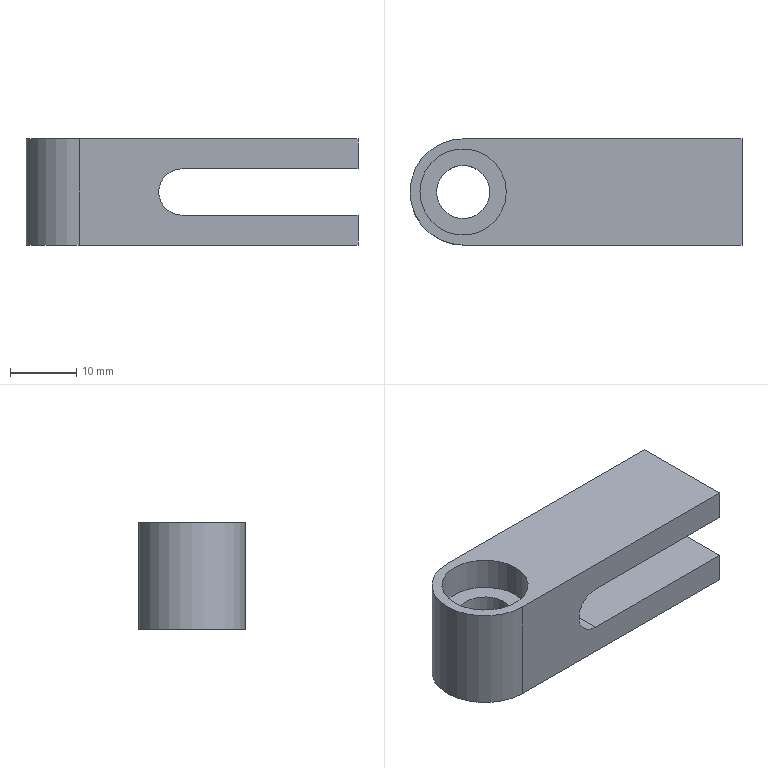CAM job | Mastercam | mm | 13 operations | part box 50 x 16 x 16
1. Facing | 24 - 100 平铣刀
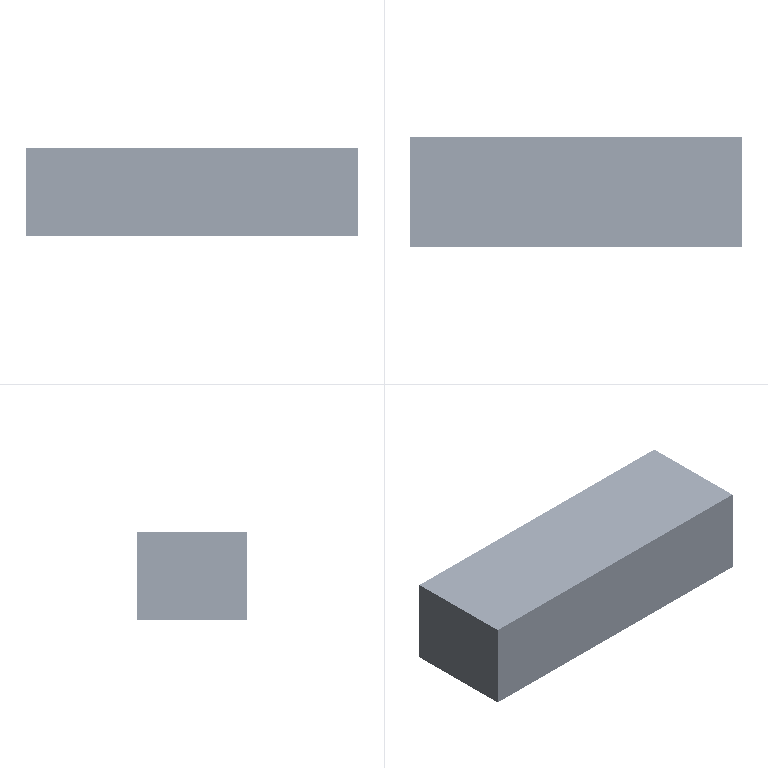2. Contour (Ramp) | 9 - 10 平铣刀
3. Contour (2D) | 10 - 10 平铣刀
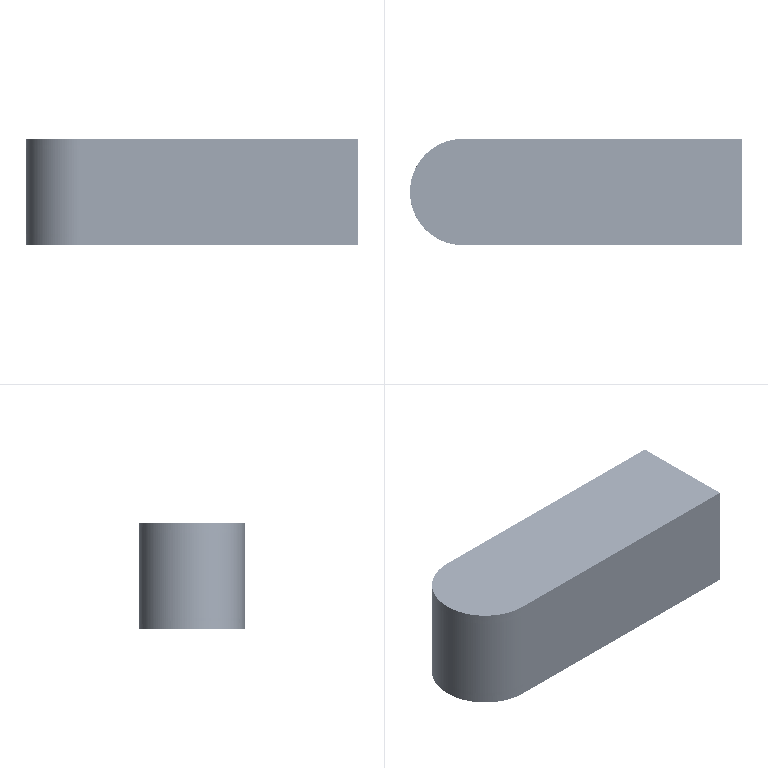4. Drill/Counterbore | 5 - 4 倒角刀
5. Peck Drill | 1 - 8 钻头
6. Contour (Ramp) | 6 - 6 平铣刀
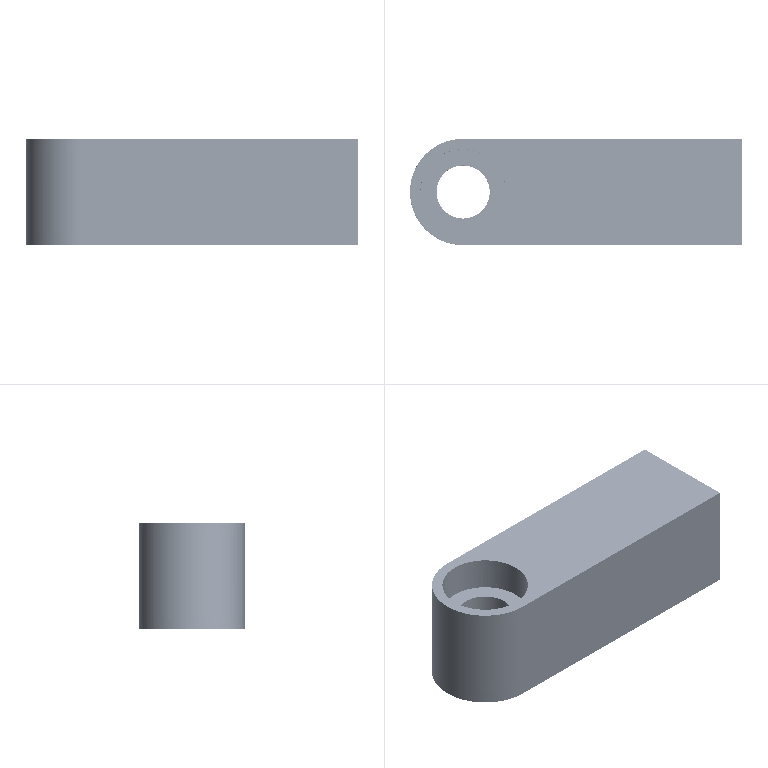7. Contour (2D) | 6 - 6 平铣刀
8. Contour (2D chamfer) | 5 - 4 倒角刀
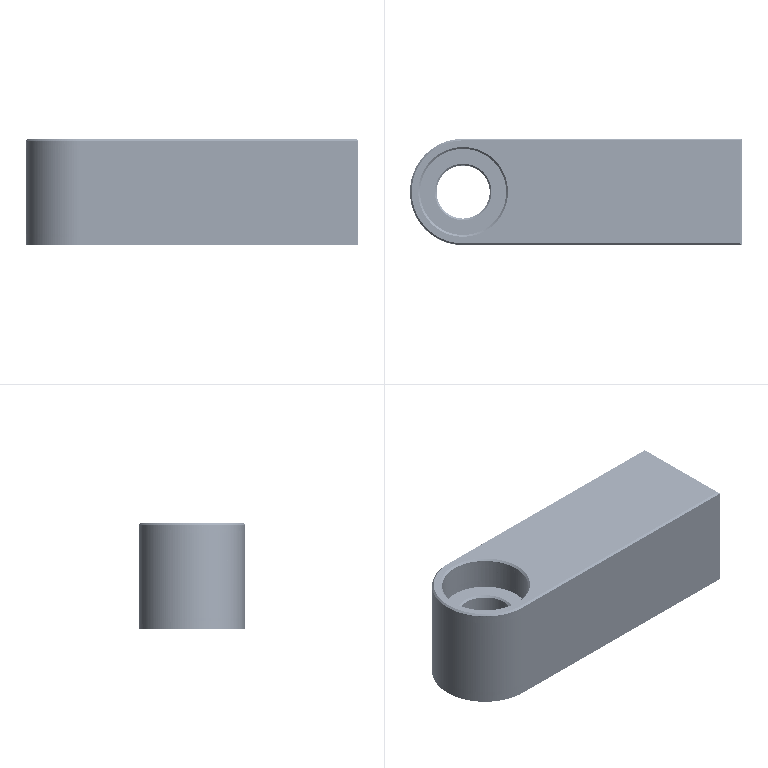9. Facing | 24 - 100 平铣刀
10. Contour (2D chamfer) | 5 - 4 倒角刀
11. Contour (Ramp) | 4 - 4 平铣刀
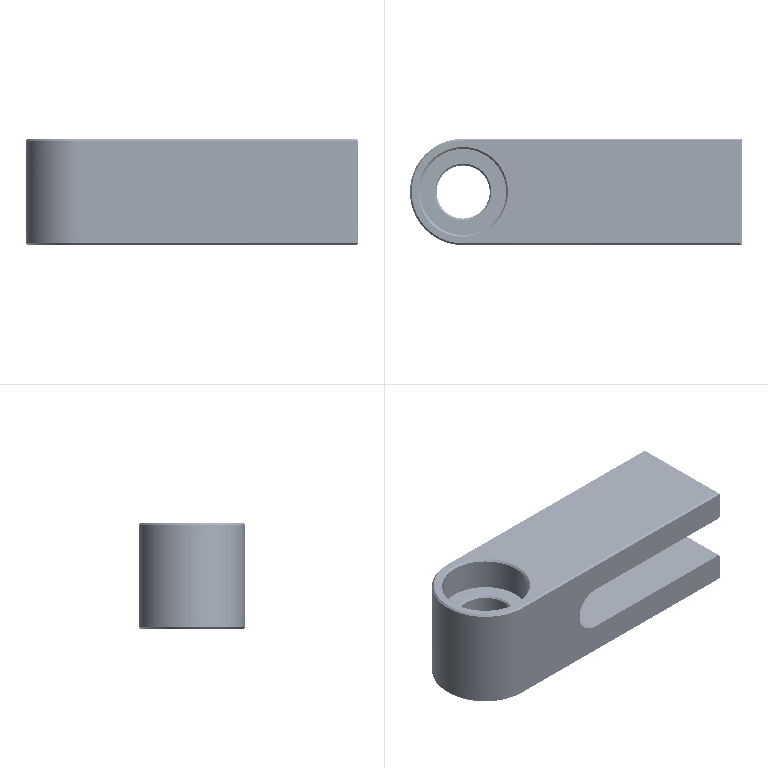12. Contour (2D) | 4 - 4 平铣刀
13. Contour (2D chamfer) | 5 - 4 倒角刀